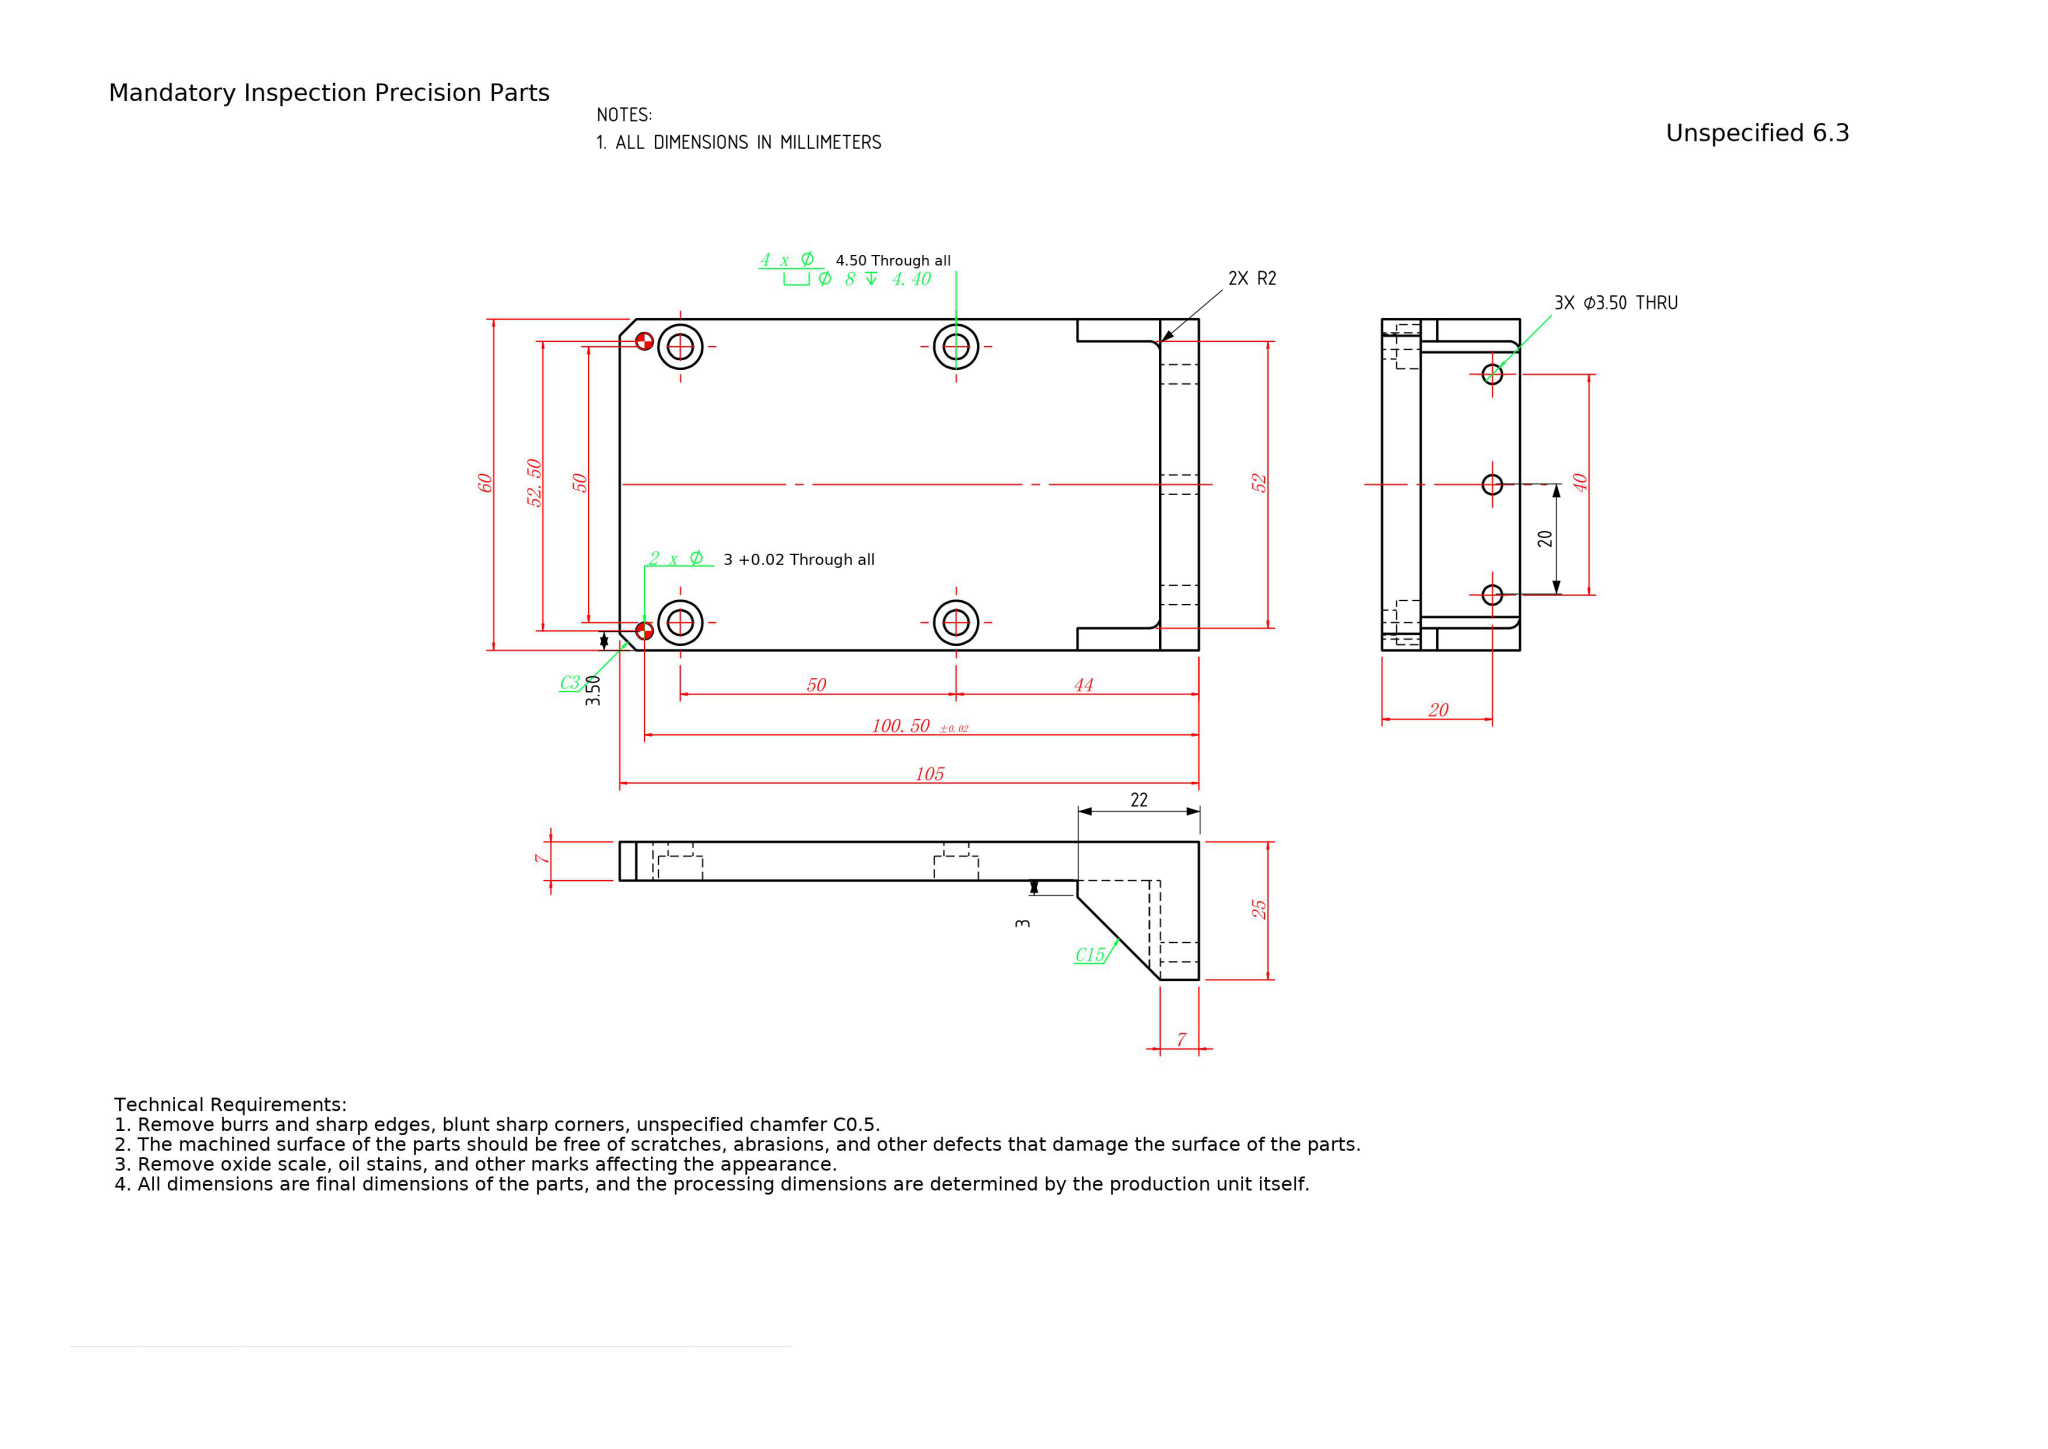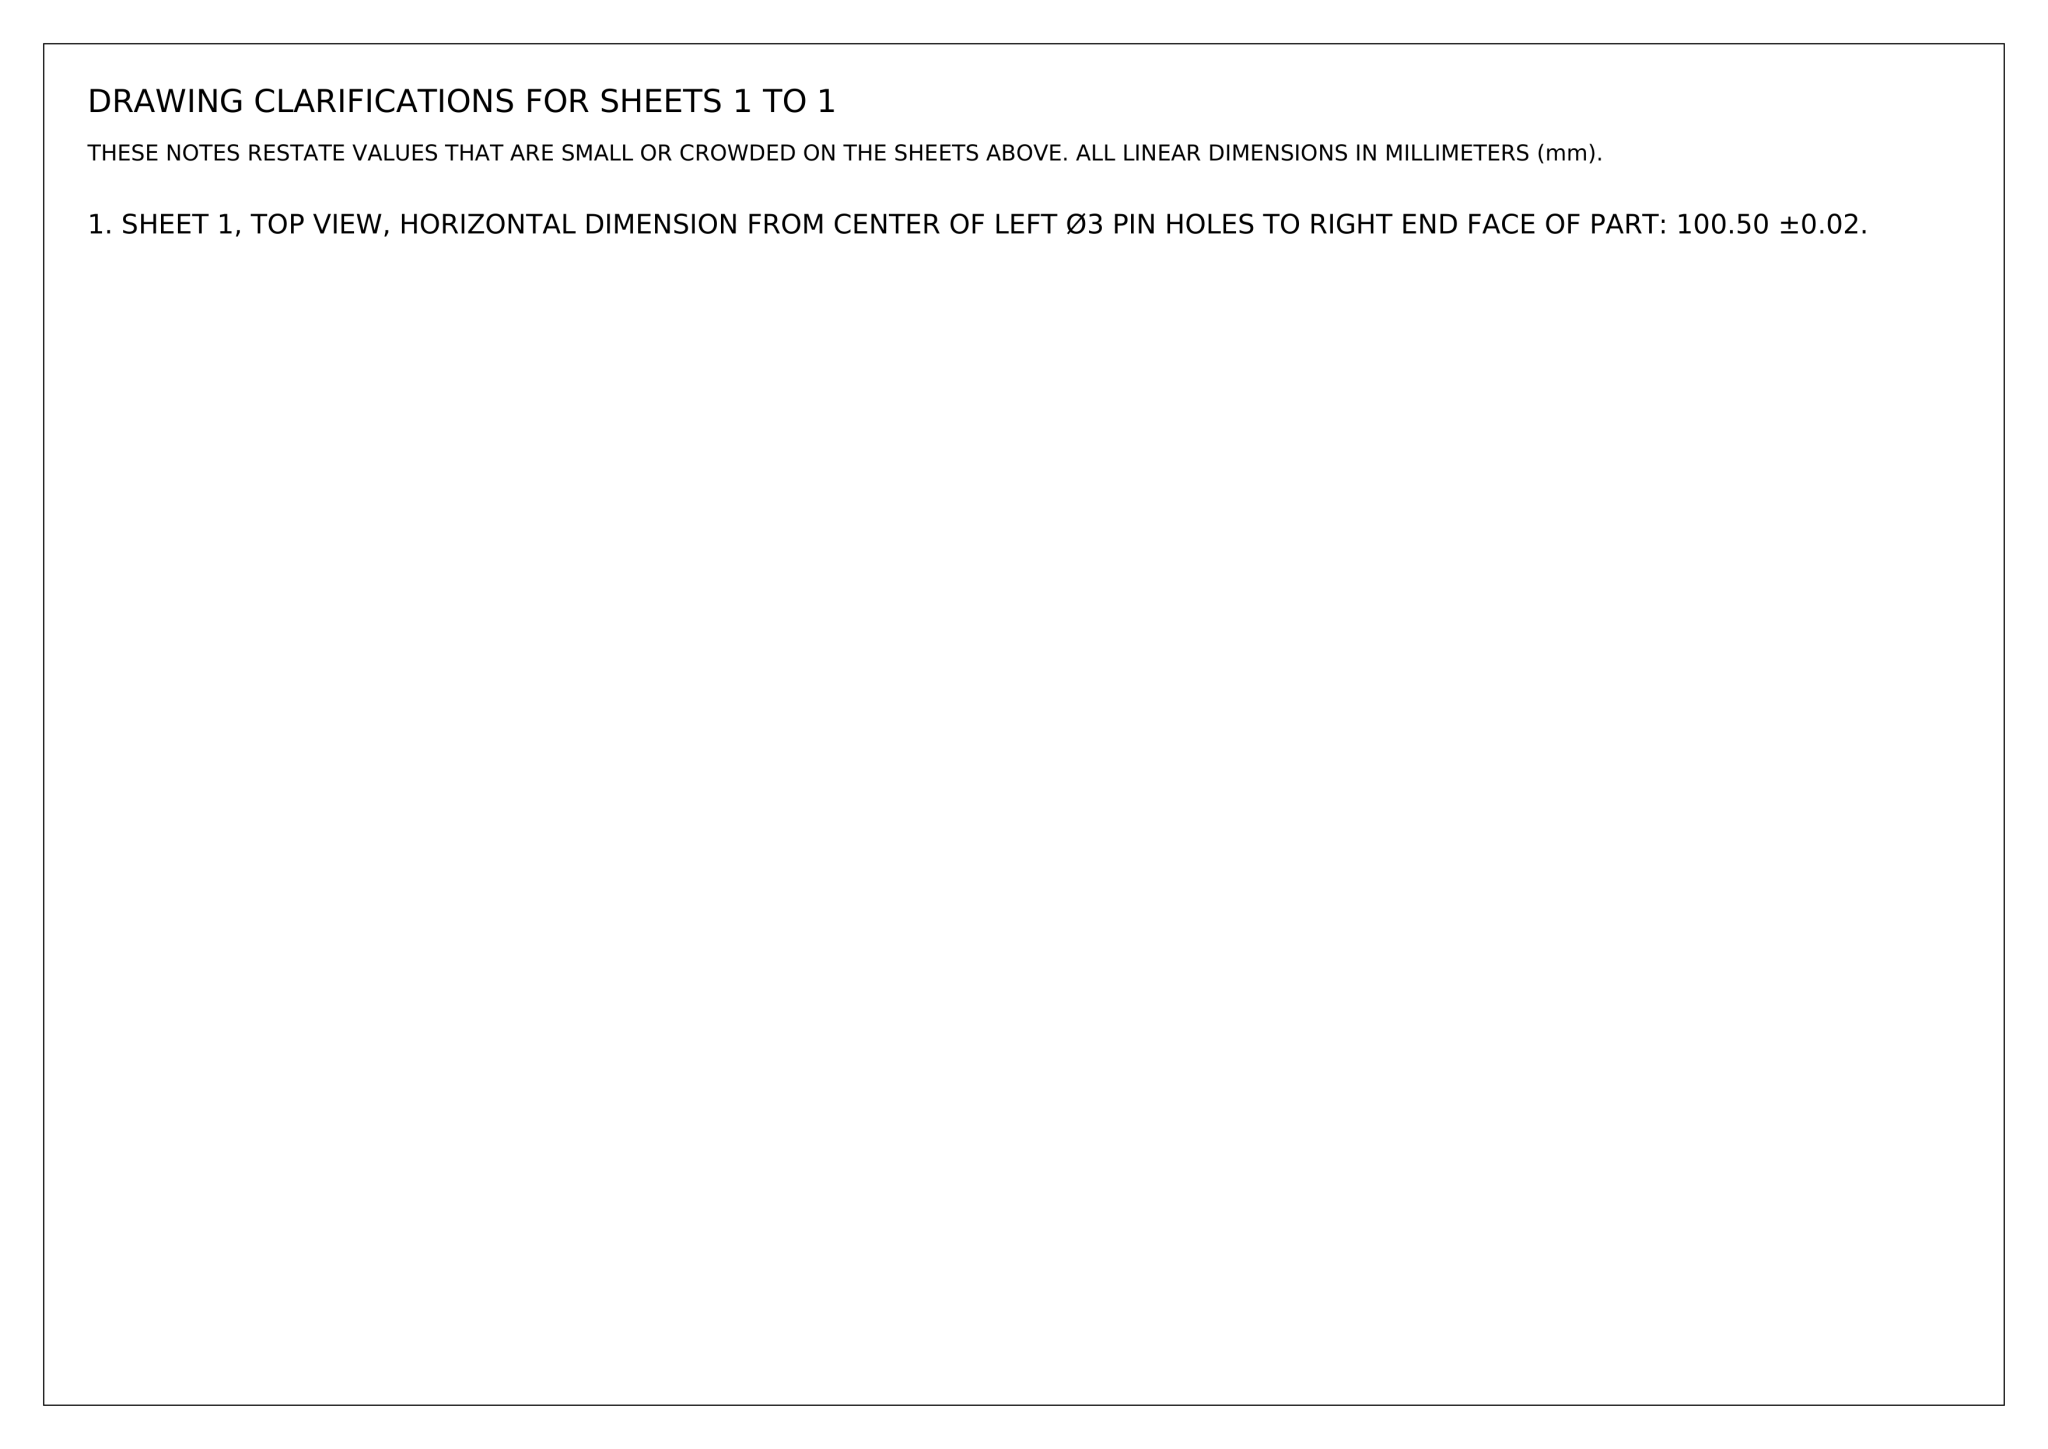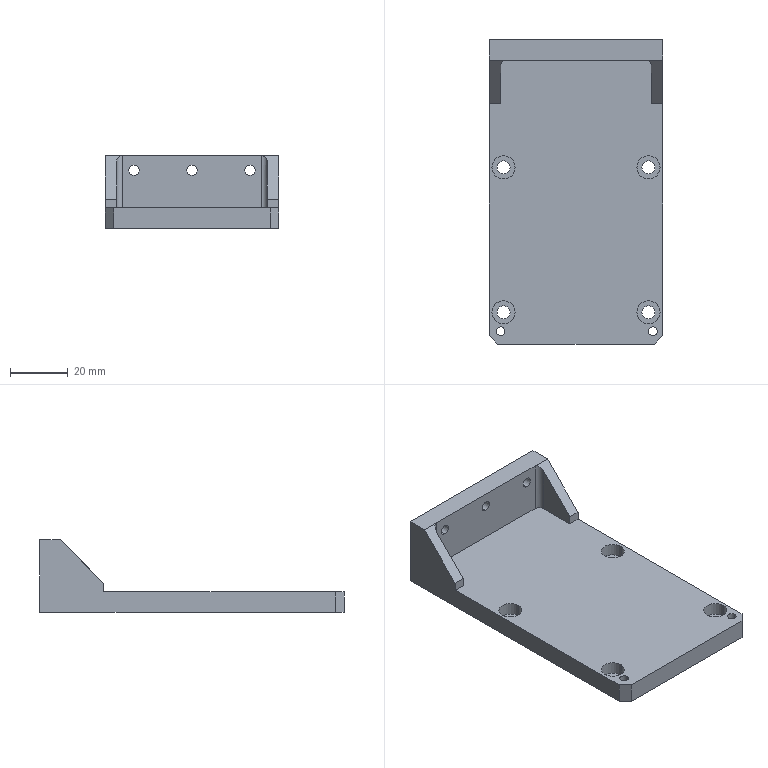Part | NX | mm | 1 solid | 48 faces | box 60 x 105 x 25 mm | volume 51536 mm3 | cylinder 28 | plane 20 | commonest cylinder face diameters 8 x8 4.5 x8 3.5 x6 3 x4 4 x2